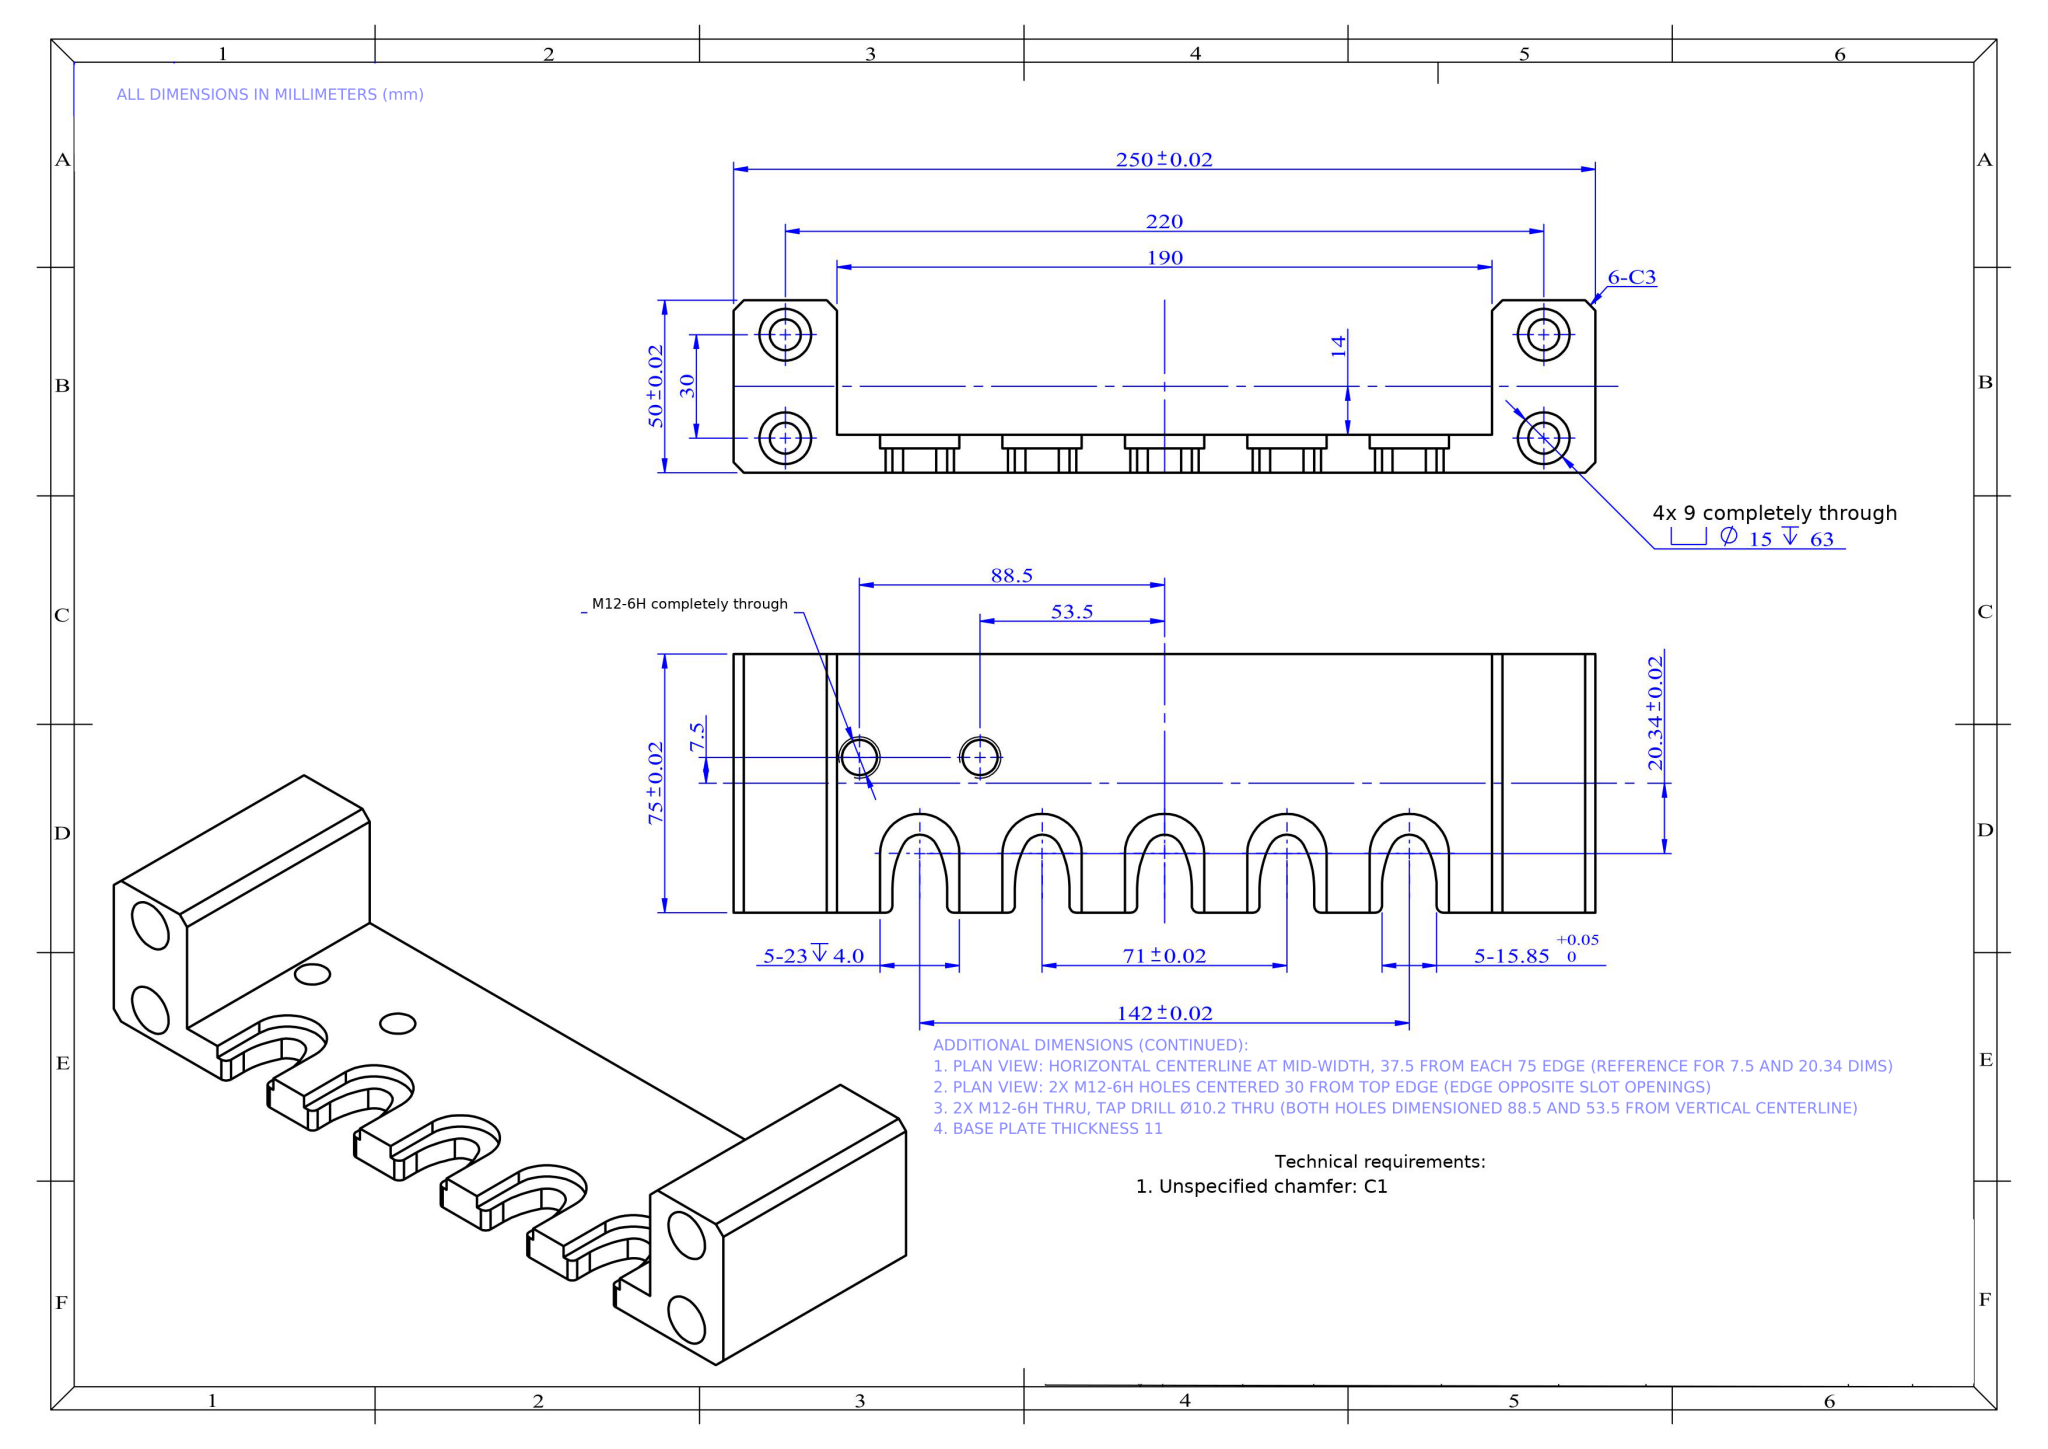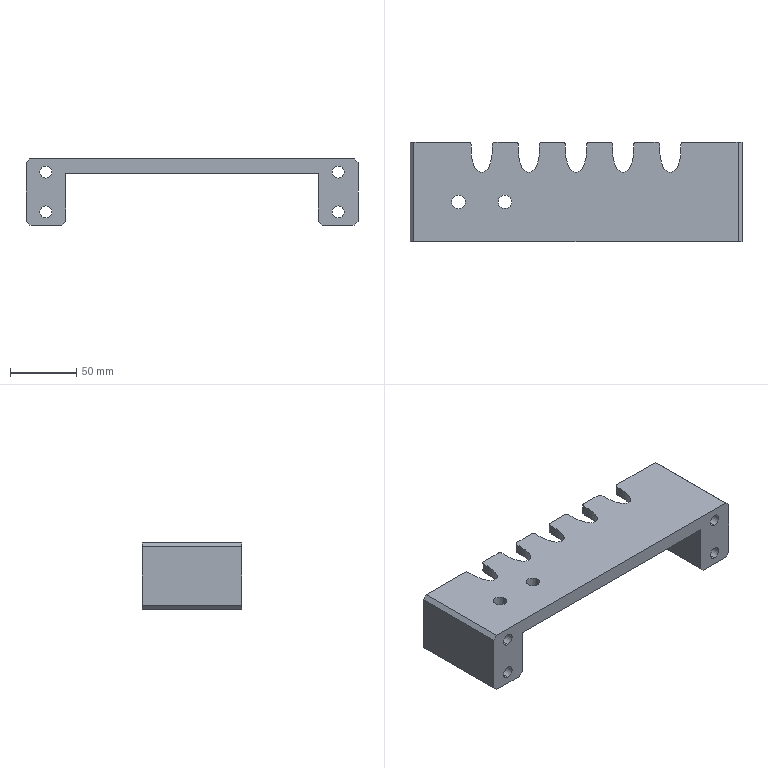Part | NX | mm | 1 solid | 100 faces | box 250 x 75 x 50 mm | volume 311101 mm3 | cylinder 50 | plane 50 | commonest cylinder face diameters 53.925 x10 4 x10 15 x8 9 x8 10.914 x5 23 x5 10.2 x4